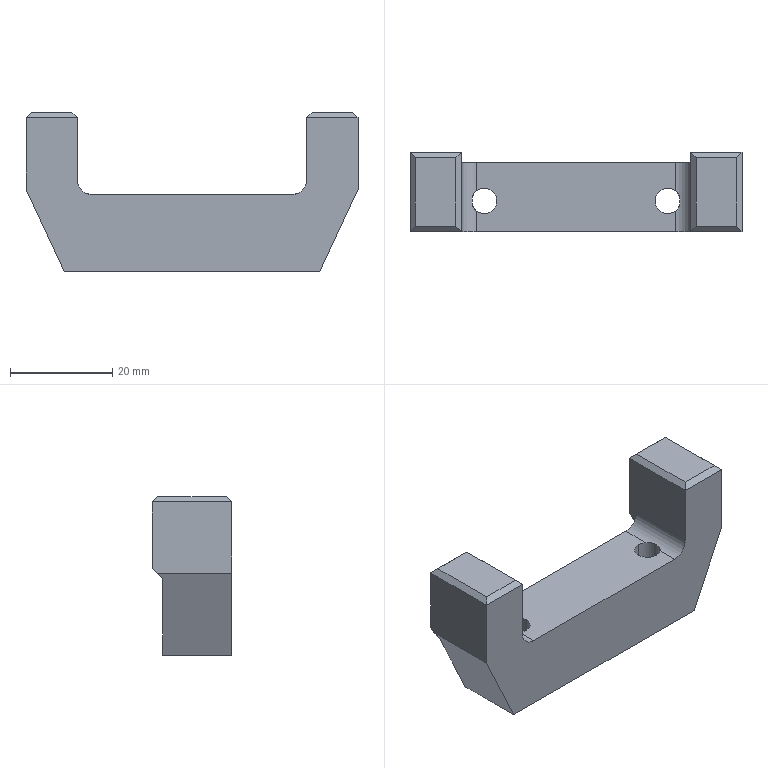Component | SolidWorks | 6.11-1937032108-0-1 | 1 solid | 40 faces | volume 15156 mm3 | plane 24 | cylinder 10 | cone 6 | commonest cylinder face diameters 6 x6 5 x4